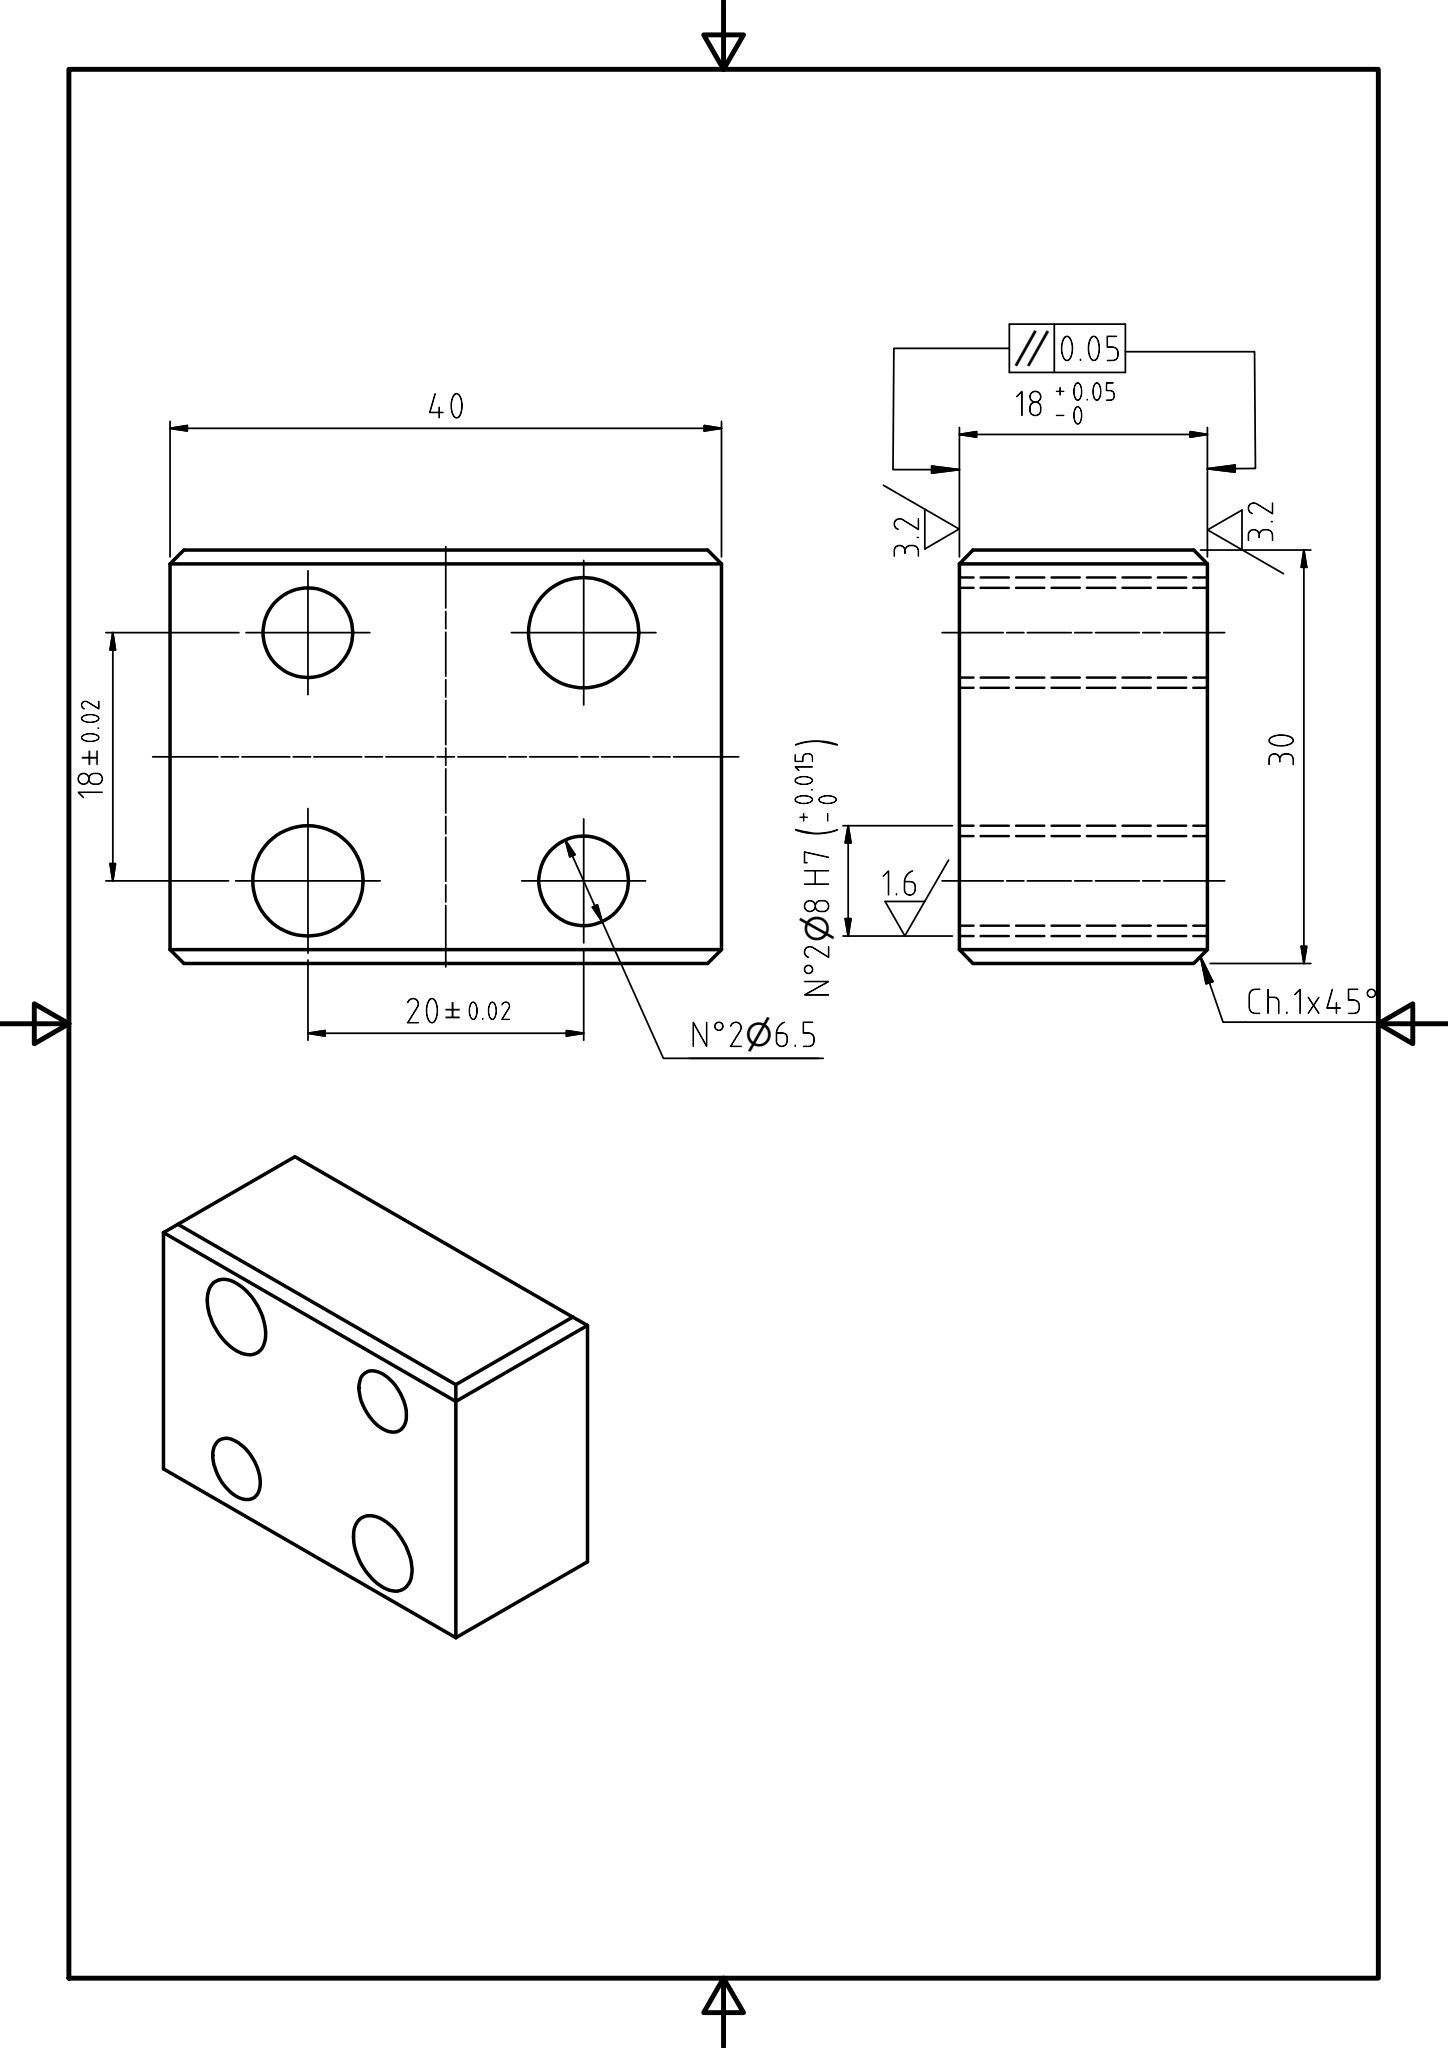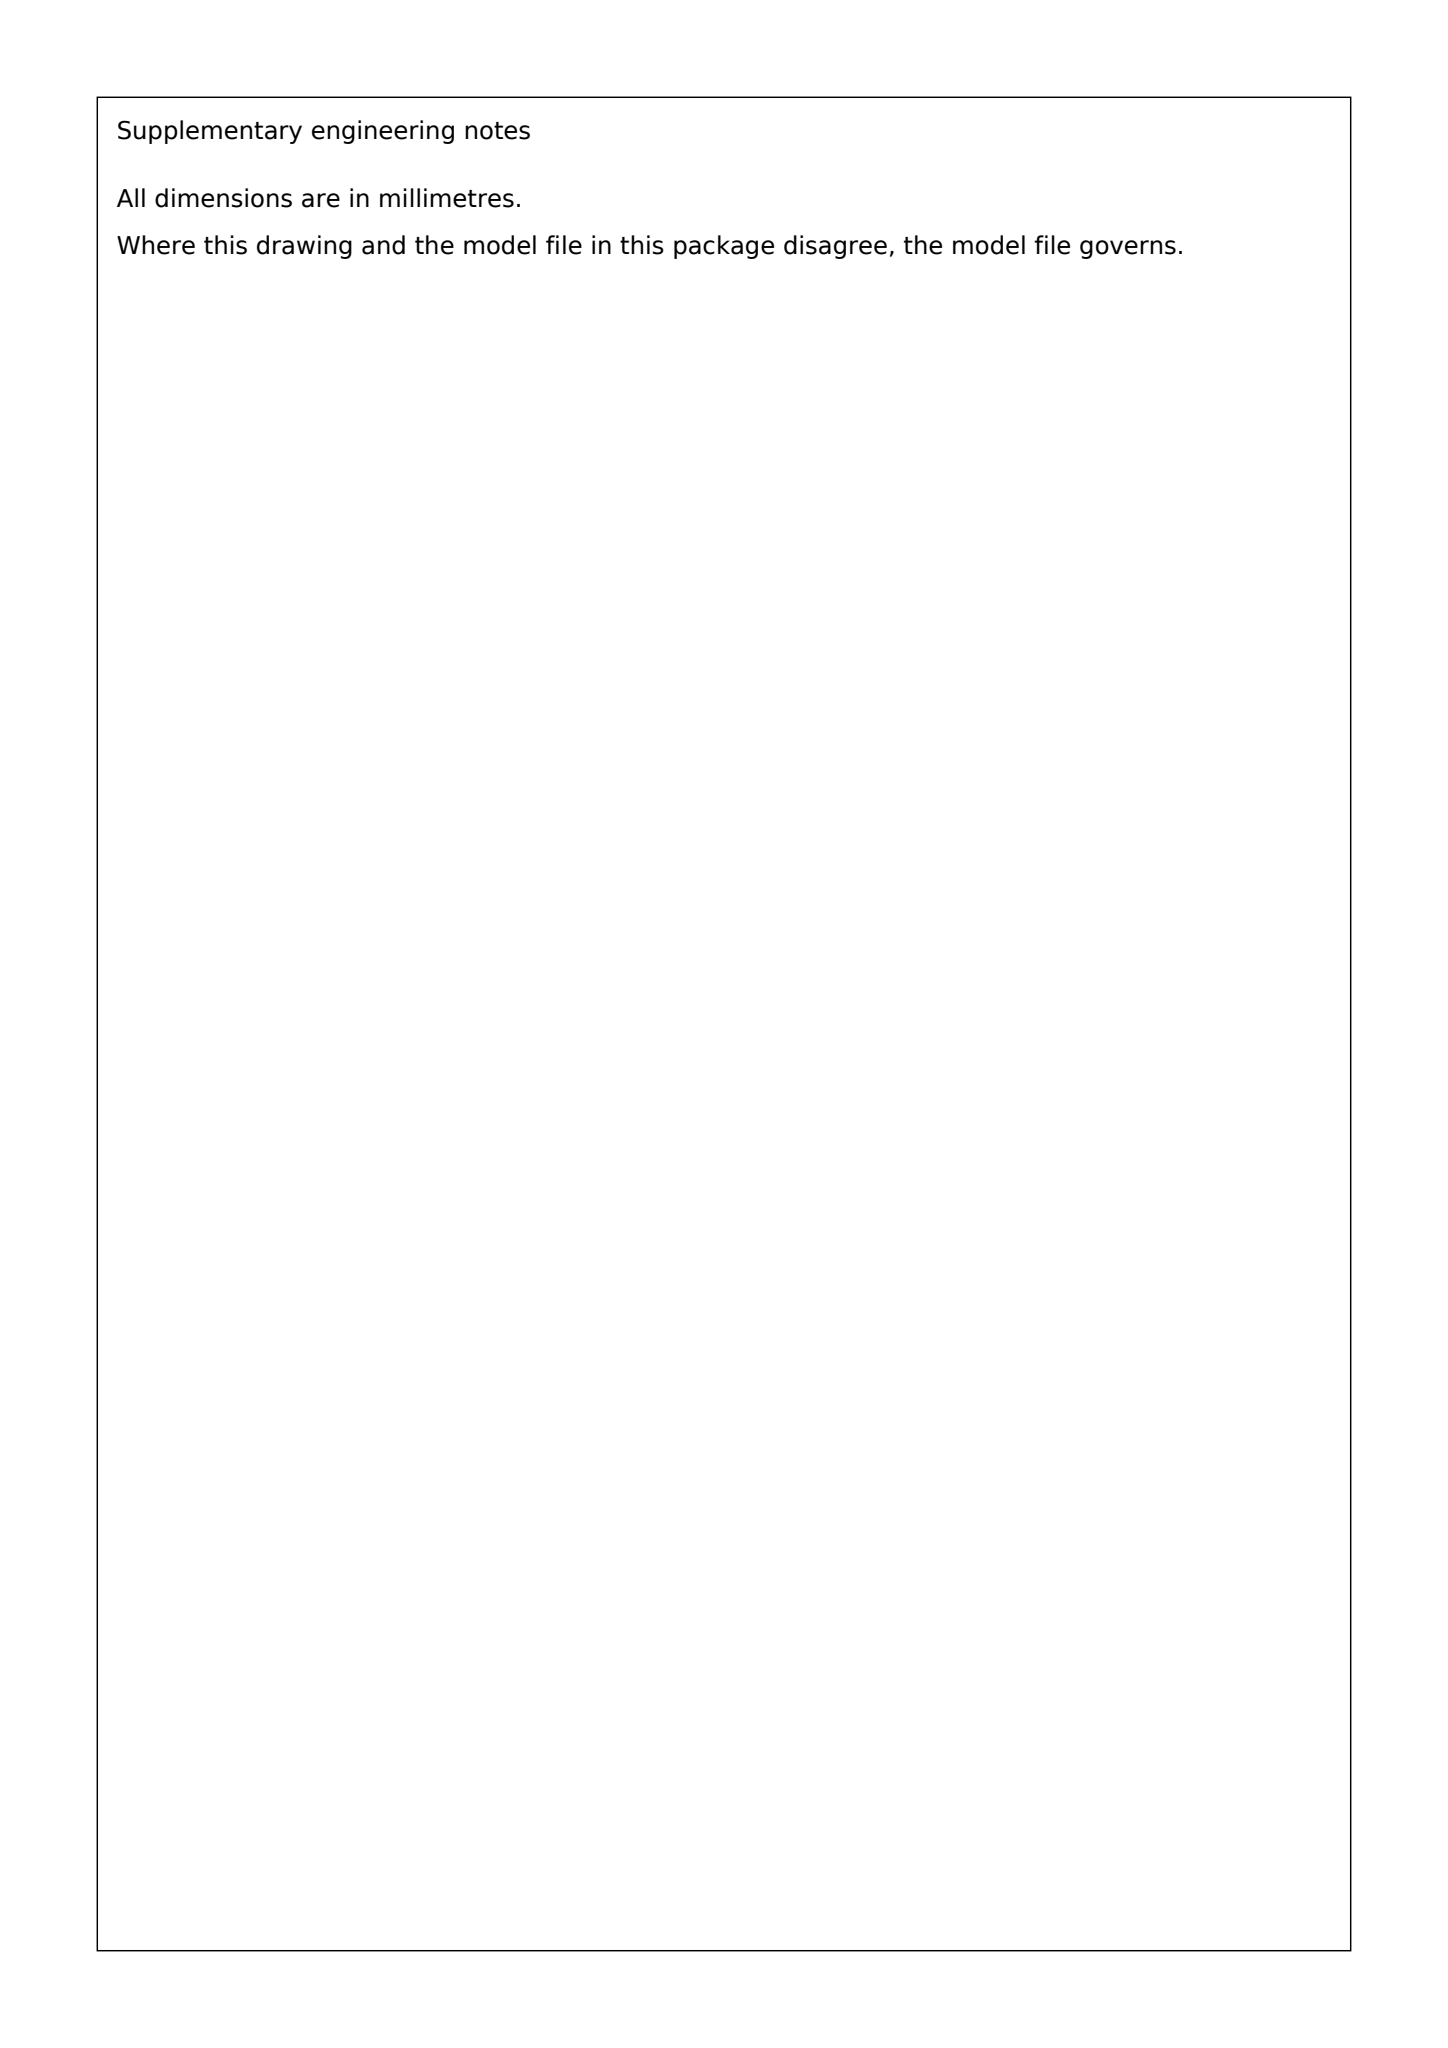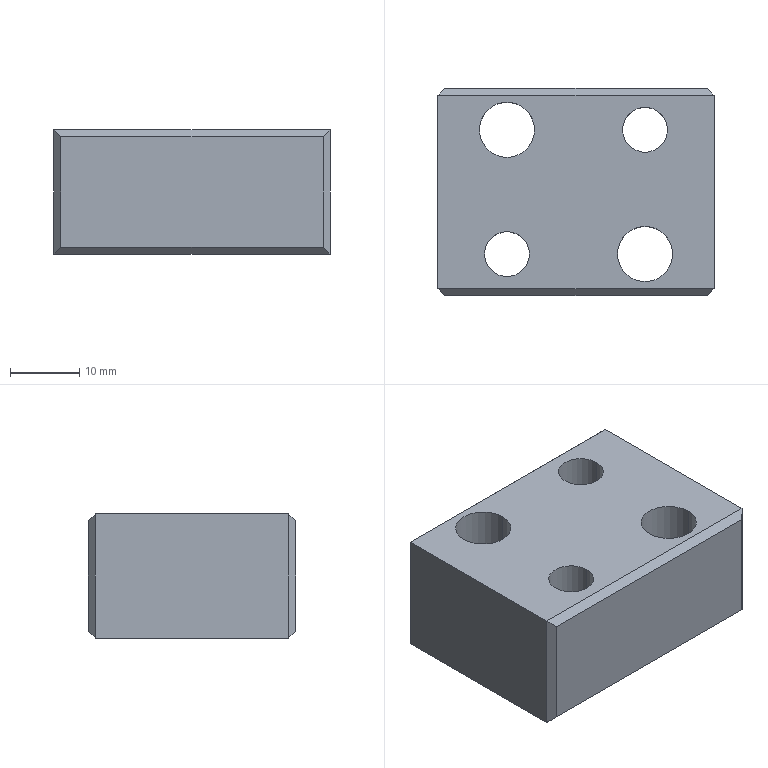Part | SolidWorks | mm | 1 solid | 22 faces | box 40 x 30 x 18 mm | volume 18483 mm3 | plane 14 | cylinder 8 | commonest cylinder face diameters 8 x4 6.5 x4
STEP:
#1=CARTESIAN_POINT('',(-14.,9.,-18.));
#2=VERTEX_POINT('',#1);
#3=CARTESIAN_POINT('',(-6.,9.,-18.));
#4=VERTEX_POINT('',#3);
#5=CARTESIAN_POINT('',(-10.,9.,-18.));
#6=DIRECTION('',(0.,0.,1.));
#7=DIRECTION('',(1.,0.,0.));
#8=AXIS2_PLACEMENT_3D('',#5,#6,#7);
#9=CIRCLE('',#8,4.);
#10=EDGE_CURVE('',#2,#4,#9,.T.);
#11=ORIENTED_EDGE('',*,*,#10,.F.);
#12=CARTESIAN_POINT('',(-14.,9.,0.));
#13=VERTEX_POINT('',#12);
#14=CARTESIAN_POINT('',(-14.,9.,-53.141));
#15=DIRECTION('',(0.,0.,1.));
#16=VECTOR('',#15,1000.);
#17=LINE('',#14,#16);
#18=EDGE_CURVE('',#2,#13,#17,.T.);
#19=ORIENTED_EDGE('',*,*,#18,.T.);
#20=CARTESIAN_POINT('',(-6.,9.,0.));
#21=VERTEX_POINT('',#20);
#22=CARTESIAN_POINT('',(-10.,9.,0.));
#23=DIRECTION('',(0.,0.,-1.));
#24=DIRECTION('',(1.,0.,0.));
#25=AXIS2_PLACEMENT_3D('',#22,#23,#24);
#26=CIRCLE('',#25,4.);
#27=EDGE_CURVE('',#21,#13,#26,.T.);
#28=ORIENTED_EDGE('',*,*,#27,.F.);
#29=CARTESIAN_POINT('',(-6.,9.,-53.141));
#30=DIRECTION('',(0.,0.,1.));
#31=VECTOR('',#30,1000.);
#32=LINE('',#29,#31);
#33=EDGE_CURVE('',#4,#21,#32,.T.);
#34=ORIENTED_EDGE('',*,*,#33,.F.);
#35=EDGE_LOOP('',(#11,#19,#28,#34));
#36=FACE_OUTER_BOUND('',#35,.T.);
#37=CARTESIAN_POINT('',(-10.,9.,-53.141));
#38=DIRECTION('',(0.,0.,1.));
#39=DIRECTION('',(1.,0.,0.));
#40=AXIS2_PLACEMENT_3D('',#37,#38,#39);
#41=CYLINDRICAL_SURFACE('',#40,4.);
#42=ADVANCED_FACE('',(#36),#41,.F.);
#43=CARTESIAN_POINT('',(6.,-9.,-18.));
#44=VERTEX_POINT('',#43);
#45=CARTESIAN_POINT('',(14.,-9.,-18.));
#46=VERTEX_POINT('',#45);
#47=CARTESIAN_POINT('',(10.,-9.,-18.));
#48=DIRECTION('',(0.,0.,1.));
#49=DIRECTION('',(1.,0.,0.));
#50=AXIS2_PLACEMENT_3D('',#47,#48,#49);
#51=CIRCLE('',#50,4.);
#52=EDGE_CURVE('',#44,#46,#51,.T.);
#53=ORIENTED_EDGE('',*,*,#52,.F.);
#54=CARTESIAN_POINT('',(6.,-9.,0.));
#55=VERTEX_POINT('',#54);
#56=CARTESIAN_POINT('',(6.,-9.,-53.141));
#57=DIRECTION('',(0.,0.,1.));
#58=VECTOR('',#57,1000.);
#59=LINE('',#56,#58);
#60=EDGE_CURVE('',#44,#55,#59,.T.);
#61=ORIENTED_EDGE('',*,*,#60,.T.);
#62=CARTESIAN_POINT('',(14.,-9.,0.));
#63=VERTEX_POINT('',#62);
#64=CARTESIAN_POINT('',(10.,-9.,0.));
#65=DIRECTION('',(0.,0.,-1.));
#66=DIRECTION('',(1.,0.,0.));
#67=AXIS2_PLACEMENT_3D('',#64,#65,#66);
#68=CIRCLE('',#67,4.);
#69=EDGE_CURVE('',#63,#55,#68,.T.);
#70=ORIENTED_EDGE('',*,*,#69,.F.);
#71=CARTESIAN_POINT('',(14.,-9.,-53.141));
#72=DIRECTION('',(0.,0.,1.));
#73=VECTOR('',#72,1000.);
#74=LINE('',#71,#73);
#75=EDGE_CURVE('',#46,#63,#74,.T.);
#76=ORIENTED_EDGE('',*,*,#75,.F.);
#77=EDGE_LOOP('',(#53,#61,#70,#76));
#78=FACE_OUTER_BOUND('',#77,.T.);
#79=CARTESIAN_POINT('',(10.,-9.,-53.141));
#80=DIRECTION('',(0.,0.,1.));
#81=DIRECTION('',(1.,0.,0.));
#82=AXIS2_PLACEMENT_3D('',#79,#80,#81);
#83=CYLINDRICAL_SURFACE('',#82,4.);
#84=ADVANCED_FACE('',(#78),#83,.F.);
#85=CARTESIAN_POINT('',(-13.25,-9.,-18.));
#86=VERTEX_POINT('',#85);
#87=CARTESIAN_POINT('',(-6.75,-9.,-18.));
#88=VERTEX_POINT('',#87);
#89=CARTESIAN_POINT('',(-10.,-9.,-18.));
#90=DIRECTION('',(0.,0.,1.));
#91=DIRECTION('',(1.,0.,0.));
#92=AXIS2_PLACEMENT_3D('',#89,#90,#91);
#93=CIRCLE('',#92,3.25);
#94=EDGE_CURVE('',#86,#88,#93,.T.);
#95=ORIENTED_EDGE('',*,*,#94,.F.);
#96=CARTESIAN_POINT('',(-13.25,-9.,0.));
#97=VERTEX_POINT('',#96);
#98=CARTESIAN_POINT('',(-13.25,-9.,-53.141));
#99=DIRECTION('',(0.,0.,1.));
#100=VECTOR('',#99,1000.);
#101=LINE('',#98,#100);
#102=EDGE_CURVE('',#86,#97,#101,.T.);
#103=ORIENTED_EDGE('',*,*,#102,.T.);
#104=CARTESIAN_POINT('',(-6.75,-9.,0.));
#105=VERTEX_POINT('',#104);
#106=CARTESIAN_POINT('',(-10.,-9.,0.));
#107=DIRECTION('',(0.,0.,-1.));
#108=DIRECTION('',(1.,0.,0.));
#109=AXIS2_PLACEMENT_3D('',#106,#107,#108);
#110=CIRCLE('',#109,3.25);
#111=EDGE_CURVE('',#105,#97,#110,.T.);
#112=ORIENTED_EDGE('',*,*,#111,.F.);
#113=CARTESIAN_POINT('',(-6.75,-9.,-53.141));
#114=DIRECTION('',(0.,0.,1.));
#115=VECTOR('',#114,1000.);
#116=LINE('',#113,#115);
#117=EDGE_CURVE('',#88,#105,#116,.T.);
#118=ORIENTED_EDGE('',*,*,#117,.F.);
#119=EDGE_LOOP('',(#95,#103,#112,#118));
#120=FACE_OUTER_BOUND('',#119,.T.);
#121=CARTESIAN_POINT('',(-10.,-9.,-53.141));
#122=DIRECTION('',(0.,0.,1.));
#123=DIRECTION('',(1.,0.,0.));
#124=AXIS2_PLACEMENT_3D('',#121,#122,#123);
#125=CYLINDRICAL_SURFACE('',#124,3.25);
#126=ADVANCED_FACE('',(#120),#125,.F.);
#127=CARTESIAN_POINT('',(6.75,9.,-18.));
#128=VERTEX_POINT('',#127);
#129=CARTESIAN_POINT('',(13.25,9.,-18.));
#130=VERTEX_POINT('',#129);
#131=CARTESIAN_POINT('',(10.,9.,-18.));
#132=DIRECTION('',(0.,0.,1.));
#133=DIRECTION('',(1.,0.,0.));
#134=AXIS2_PLACEMENT_3D('',#131,#132,#133);
#135=CIRCLE('',#134,3.25);
#136=EDGE_CURVE('',#128,#130,#135,.T.);
#137=ORIENTED_EDGE('',*,*,#136,.F.);
#138=CARTESIAN_POINT('',(6.75,9.,0.));
#139=VERTEX_POINT('',#138);
#140=CARTESIAN_POINT('',(6.75,9.,-53.141));
#141=DIRECTION('',(0.,0.,1.));
#142=VECTOR('',#141,1000.);
#143=LINE('',#140,#142);
#144=EDGE_CURVE('',#128,#139,#143,.T.);
#145=ORIENTED_EDGE('',*,*,#144,.T.);
#146=CARTESIAN_POINT('',(13.25,9.,0.));
#147=VERTEX_POINT('',#146);
#148=CARTESIAN_POINT('',(10.,9.,0.));
#149=DIRECTION('',(0.,0.,-1.));
#150=DIRECTION('',(1.,0.,0.));
#151=AXIS2_PLACEMENT_3D('',#148,#149,#150);
#152=CIRCLE('',#151,3.25);
#153=EDGE_CURVE('',#147,#139,#152,.T.);
#154=ORIENTED_EDGE('',*,*,#153,.F.);
#155=CARTESIAN_POINT('',(13.25,9.,-53.141));
#156=DIRECTION('',(0.,0.,1.));
#157=VECTOR('',#156,1000.);
#158=LINE('',#155,#157);
#159=EDGE_CURVE('',#130,#147,#158,.T.);
#160=ORIENTED_EDGE('',*,*,#159,.F.);
#161=EDGE_LOOP('',(#137,#145,#154,#160));
#162=FACE_OUTER_BOUND('',#161,.T.);
#163=CARTESIAN_POINT('',(10.,9.,-53.141));
#164=DIRECTION('',(0.,0.,1.));
#165=DIRECTION('',(1.,0.,0.));
#166=AXIS2_PLACEMENT_3D('',#163,#164,#165);
#167=CYLINDRICAL_SURFACE('',#166,3.25);
#168=ADVANCED_FACE('',(#162),#167,.F.);
#169=CARTESIAN_POINT('',(20.,-14.,0.));
#170=VERTEX_POINT('',#169);
#171=CARTESIAN_POINT('',(-20.,-14.,0.));
#172=VERTEX_POINT('',#171);
#173=CARTESIAN_POINT('',(-10.,-14.,0.));
#174=DIRECTION('',(-1.,-0.,0.));
#175=VECTOR('',#174,1000.);
#176=LINE('',#173,#175);
#177=EDGE_CURVE('',#170,#172,#176,.T.);
#178=ORIENTED_EDGE('',*,*,#177,.T.);
#179=CARTESIAN_POINT('',(-19.,-15.,-1.));
#180=VERTEX_POINT('',#179);
#181=CARTESIAN_POINT('',(-20.,-14.,0.));
#182=DIRECTION('',(0.5774,-0.5774,-0.5774));
#183=VECTOR('',#182,1000.);
#184=LINE('',#181,#183);
#185=EDGE_CURVE('',#172,#180,#184,.T.);
#186=ORIENTED_EDGE('',*,*,#185,.T.);
#187=CARTESIAN_POINT('',(19.,-15.,-1.));
#188=VERTEX_POINT('',#187);
#189=CARTESIAN_POINT('',(-10.,-15.,-1.));
#190=DIRECTION('',(1.,0.,0.));
#191=VECTOR('',#190,1000.);
#192=LINE('',#189,#191);
#193=EDGE_CURVE('',#180,#188,#192,.T.);
#194=ORIENTED_EDGE('',*,*,#193,.T.);
#195=CARTESIAN_POINT('',(19.,-15.,-1.));
#196=DIRECTION('',(0.5774,0.5774,0.5774));
#197=VECTOR('',#196,1000.);
#198=LINE('',#195,#197);
#199=EDGE_CURVE('',#188,#170,#198,.T.);
#200=ORIENTED_EDGE('',*,*,#199,.T.);
#201=EDGE_LOOP('',(#178,#186,#194,#200));
#202=FACE_OUTER_BOUND('',#201,.T.);
#203=CARTESIAN_POINT('',(-10.,-14.5,-0.5));
#204=DIRECTION('',(0.,-0.7071,0.7071));
#205=DIRECTION('',(-1.,-0.,0.));
#206=AXIS2_PLACEMENT_3D('',#203,#204,#205);
#207=PLANE('',#206);
#208=ADVANCED_FACE('',(#202),#207,.T.);
#209=CARTESIAN_POINT('',(19.,-15.,-17.));
#210=VERTEX_POINT('',#209);
#211=CARTESIAN_POINT('',(19.,-15.,0.));
#212=DIRECTION('',(0.,0.,-1.));
#213=VECTOR('',#212,1000.);
#214=LINE('',#211,#213);
#215=EDGE_CURVE('',#188,#210,#214,.T.);
#216=ORIENTED_EDGE('',*,*,#215,.T.);
#217=CARTESIAN_POINT('',(20.,-14.,-18.));
#218=VERTEX_POINT('',#217);
#219=CARTESIAN_POINT('',(19.,-15.,-17.));
#220=DIRECTION('',(0.5774,0.5774,-0.5774));
#221=VECTOR('',#220,1000.);
#222=LINE('',#219,#221);
#223=EDGE_CURVE('',#210,#218,#222,.T.);
#224=ORIENTED_EDGE('',*,*,#223,.T.);
#225=CARTESIAN_POINT('',(20.,-14.,0.));
#226=DIRECTION('',(0.,0.,1.));
#227=VECTOR('',#226,1000.);
#228=LINE('',#225,#227);
#229=EDGE_CURVE('',#218,#170,#228,.T.);
#230=ORIENTED_EDGE('',*,*,#229,.T.);
#231=ORIENTED_EDGE('',*,*,#199,.F.);
#232=EDGE_LOOP('',(#216,#224,#230,#231));
#233=FACE_OUTER_BOUND('',#232,.T.);
#234=CARTESIAN_POINT('',(19.5,-14.5,0.));
#235=DIRECTION('',(0.7071,-0.7071,0.));
#236=DIRECTION('',(0.,0.,-1.));
#237=AXIS2_PLACEMENT_3D('',#234,#235,#236);
#238=PLANE('',#237);
#239=ADVANCED_FACE('',(#233),#238,.T.);
#240=CARTESIAN_POINT('',(-20.,-14.,-18.));
#241=VERTEX_POINT('',#240);
#242=CARTESIAN_POINT('',(-10.,-14.,-18.));
#243=DIRECTION('',(1.,0.,0.));
#244=VECTOR('',#243,1000.);
#245=LINE('',#242,#244);
#246=EDGE_CURVE('',#241,#218,#245,.T.);
#247=ORIENTED_EDGE('',*,*,#246,.T.);
#248=ORIENTED_EDGE('',*,*,#223,.F.);
#249=CARTESIAN_POINT('',(-19.,-15.,-17.));
#250=VERTEX_POINT('',#249);
#251=CARTESIAN_POINT('',(-10.,-15.,-17.));
#252=DIRECTION('',(-1.,-0.,0.));
#253=VECTOR('',#252,1000.);
#254=LINE('',#251,#253);
#255=EDGE_CURVE('',#210,#250,#254,.T.);
#256=ORIENTED_EDGE('',*,*,#255,.T.);
#257=CARTESIAN_POINT('',(-20.,-14.,-18.));
#258=DIRECTION('',(0.5774,-0.5774,0.5774));
#259=VECTOR('',#258,1000.);
#260=LINE('',#257,#259);
#261=EDGE_CURVE('',#241,#250,#260,.T.);
#262=ORIENTED_EDGE('',*,*,#261,.F.);
#263=EDGE_LOOP('',(#247,#248,#256,#262));
#264=FACE_OUTER_BOUND('',#263,.T.);
#265=CARTESIAN_POINT('',(-10.,-14.5,-17.5));
#266=DIRECTION('',(0.,-0.7071,-0.7071));
#267=DIRECTION('',(0.,-0.7071,0.7071));
#268=AXIS2_PLACEMENT_3D('',#265,#266,#267);
#269=PLANE('',#268);
#270=ADVANCED_FACE('',(#264),#269,.T.);
#271=CARTESIAN_POINT('',(-20.,-14.,0.));
#272=DIRECTION('',(0.,0.,-1.));
#273=VECTOR('',#272,1000.);
#274=LINE('',#271,#273);
#275=EDGE_CURVE('',#172,#241,#274,.T.);
#276=ORIENTED_EDGE('',*,*,#275,.T.);
#277=ORIENTED_EDGE('',*,*,#261,.T.);
#278=CARTESIAN_POINT('',(-19.,-15.,0.));
#279=DIRECTION('',(0.,0.,1.));
#280=VECTOR('',#279,1000.);
#281=LINE('',#278,#280);
#282=EDGE_CURVE('',#250,#180,#281,.T.);
#283=ORIENTED_EDGE('',*,*,#282,.T.);
#284=ORIENTED_EDGE('',*,*,#185,.F.);
#285=EDGE_LOOP('',(#276,#277,#283,#284));
#286=FACE_OUTER_BOUND('',#285,.T.);
#287=CARTESIAN_POINT('',(-19.5,-14.5,0.));
#288=DIRECTION('',(-0.7071,-0.7071,0.));
#289=DIRECTION('',(-0.7071,0.7071,0.));
#290=AXIS2_PLACEMENT_3D('',#287,#288,#289);
#291=PLANE('',#290);
#292=ADVANCED_FACE('',(#286),#291,.T.);
#293=ORIENTED_EDGE('',*,*,#275,.F.);
#294=CARTESIAN_POINT('',(-20.,14.,0.));
#295=VERTEX_POINT('',#294);
#296=CARTESIAN_POINT('',(-20.,-15.,0.));
#297=DIRECTION('',(0.,1.,0.));
#298=VECTOR('',#297,1000.);
#299=LINE('',#296,#298);
#300=EDGE_CURVE('',#172,#295,#299,.T.);
#301=ORIENTED_EDGE('',*,*,#300,.T.);
#302=CARTESIAN_POINT('',(-20.,14.,-18.));
#303=VERTEX_POINT('',#302);
#304=CARTESIAN_POINT('',(-20.,14.,0.));
#305=DIRECTION('',(0.,0.,1.));
#306=VECTOR('',#305,1000.);
#307=LINE('',#304,#306);
#308=EDGE_CURVE('',#303,#295,#307,.T.);
#309=ORIENTED_EDGE('',*,*,#308,.F.);
#310=CARTESIAN_POINT('',(-20.,-15.,-18.));
#311=DIRECTION('',(0.,-1.,0.));
#312=VECTOR('',#311,1000.);
#313=LINE('',#310,#312);
#314=EDGE_CURVE('',#303,#241,#313,.T.);
#315=ORIENTED_EDGE('',*,*,#314,.T.);
#316=EDGE_LOOP('',(#293,#301,#309,#315));
#317=FACE_OUTER_BOUND('',#316,.T.);
#318=CARTESIAN_POINT('',(-20.,15.,0.));
#319=DIRECTION('',(-1.,0.,0.));
#320=DIRECTION('',(0.,0.,1.));
#321=AXIS2_PLACEMENT_3D('',#318,#319,#320);
#322=PLANE('',#321);
#323=ADVANCED_FACE('',(#317),#322,.T.);
#324=ORIENTED_EDGE('',*,*,#177,.F.);
#325=CARTESIAN_POINT('',(20.,14.,0.));
#326=VERTEX_POINT('',#325);
#327=CARTESIAN_POINT('',(20.,15.,0.));
#328=DIRECTION('',(0.,-1.,0.));
#329=VECTOR('',#328,1000.);
#330=LINE('',#327,#329);
#331=EDGE_CURVE('',#326,#170,#330,.T.);
#332=ORIENTED_EDGE('',*,*,#331,.F.);
#333=CARTESIAN_POINT('',(10.,14.,0.));
#334=DIRECTION('',(1.,-0.,0.));
#335=VECTOR('',#334,1000.);
#336=LINE('',#333,#335);
#337=EDGE_CURVE('',#295,#326,#336,.T.);
#338=ORIENTED_EDGE('',*,*,#337,.F.);
#339=ORIENTED_EDGE('',*,*,#300,.F.);
#340=EDGE_LOOP('',(#324,#332,#338,#339));
#341=FACE_OUTER_BOUND('',#340,.T.);
#342=ORIENTED_EDGE('',*,*,#153,.T.);
#343=CARTESIAN_POINT('',(10.,9.,0.));
#344=DIRECTION('',(0.,0.,-1.));
#345=DIRECTION('',(1.,0.,0.));
#346=AXIS2_PLACEMENT_3D('',#343,#344,#345);
#347=CIRCLE('',#346,3.25);
#348=EDGE_CURVE('',#139,#147,#347,.T.);
#349=ORIENTED_EDGE('',*,*,#348,.T.);
#350=EDGE_LOOP('',(#342,#349));
#351=FACE_BOUND('',#350,.T.);
#352=ORIENTED_EDGE('',*,*,#111,.T.);
#353=CARTESIAN_POINT('',(-10.,-9.,0.));
#354=DIRECTION('',(0.,0.,-1.));
#355=DIRECTION('',(1.,0.,0.));
#356=AXIS2_PLACEMENT_3D('',#353,#354,#355);
#357=CIRCLE('',#356,3.25);
#358=EDGE_CURVE('',#97,#105,#357,.T.);
#359=ORIENTED_EDGE('',*,*,#358,.T.);
#360=EDGE_LOOP('',(#352,#359));
#361=FACE_BOUND('',#360,.T.);
#362=ORIENTED_EDGE('',*,*,#69,.T.);
#363=CARTESIAN_POINT('',(10.,-9.,0.));
#364=DIRECTION('',(0.,0.,-1.));
#365=DIRECTION('',(1.,0.,0.));
#366=AXIS2_PLACEMENT_3D('',#363,#364,#365);
#367=CIRCLE('',#366,4.);
#368=EDGE_CURVE('',#55,#63,#367,.T.);
#369=ORIENTED_EDGE('',*,*,#368,.T.);
#370=EDGE_LOOP('',(#362,#369));
#371=FACE_BOUND('',#370,.T.);
#372=ORIENTED_EDGE('',*,*,#27,.T.);
#373=CARTESIAN_POINT('',(-10.,9.,0.));
#374=DIRECTION('',(0.,0.,-1.));
#375=DIRECTION('',(1.,0.,0.));
#376=AXIS2_PLACEMENT_3D('',#373,#374,#375);
#377=CIRCLE('',#376,4.);
#378=EDGE_CURVE('',#13,#21,#377,.T.);
#379=ORIENTED_EDGE('',*,*,#378,.T.);
#380=EDGE_LOOP('',(#372,#379));
#381=FACE_BOUND('',#380,.T.);
#382=CARTESIAN_POINT('',(0.,0.,0.));
#383=DIRECTION('',(0.,0.,1.));
#384=DIRECTION('',(1.,0.,0.));
#385=AXIS2_PLACEMENT_3D('',#382,#383,#384);
#386=PLANE('',#385);
#387=ADVANCED_FACE('',(#341,#351,#361,#371,#381),#386,.T.);
#388=ORIENTED_EDGE('',*,*,#193,.F.);
#389=ORIENTED_EDGE('',*,*,#282,.F.);
#390=ORIENTED_EDGE('',*,*,#255,.F.);
#391=ORIENTED_EDGE('',*,*,#215,.F.);
#392=EDGE_LOOP('',(#388,#389,#390,#391));
#393=FACE_OUTER_BOUND('',#392,.T.);
#394=CARTESIAN_POINT('',(-20.,-15.,0.));
#395=DIRECTION('',(0.,-1.,0.));
#396=DIRECTION('',(0.,0.,-1.));
#397=AXIS2_PLACEMENT_3D('',#394,#395,#396);
#398=PLANE('',#397);
#399=ADVANCED_FACE('',(#393),#398,.T.);
#400=ORIENTED_EDGE('',*,*,#337,.T.);
#401=CARTESIAN_POINT('',(19.,15.,-1.));
#402=VERTEX_POINT('',#401);
#403=CARTESIAN_POINT('',(20.,14.,0.));
#404=DIRECTION('',(-0.5774,0.5774,-0.5774));
#405=VECTOR('',#404,1000.);
#406=LINE('',#403,#405);
#407=EDGE_CURVE('',#326,#402,#406,.T.);
#408=ORIENTED_EDGE('',*,*,#407,.T.);
#409=CARTESIAN_POINT('',(-19.,15.,-1.));
#410=VERTEX_POINT('',#409);
#411=CARTESIAN_POINT('',(10.,15.,-1.));
#412=DIRECTION('',(-1.,0.,0.));
#413=VECTOR('',#412,1000.);
#414=LINE('',#411,#413);
#415=EDGE_CURVE('',#402,#410,#414,.T.);
#416=ORIENTED_EDGE('',*,*,#415,.T.);
#417=CARTESIAN_POINT('',(-19.,15.,-1.));
#418=DIRECTION('',(-0.5774,-0.5774,0.5774));
#419=VECTOR('',#418,1000.);
#420=LINE('',#417,#419);
#421=EDGE_CURVE('',#410,#295,#420,.T.);
#422=ORIENTED_EDGE('',*,*,#421,.T.);
#423=EDGE_LOOP('',(#400,#408,#416,#422));
#424=FACE_OUTER_BOUND('',#423,.T.);
#425=CARTESIAN_POINT('',(10.,14.5,-0.5));
#426=DIRECTION('',(0.,0.7071,0.7071));
#427=DIRECTION('',(1.,-0.,0.));
#428=AXIS2_PLACEMENT_3D('',#425,#426,#427);
#429=PLANE('',#428);
#430=ADVANCED_FACE('',(#424),#429,.T.);
#431=CARTESIAN_POINT('',(-19.,15.,-17.));
#432=VERTEX_POINT('',#431);
#433=CARTESIAN_POINT('',(-19.,15.,0.));
#434=DIRECTION('',(0.,0.,-1.));
#435=VECTOR('',#434,1000.);
#436=LINE('',#433,#435);
#437=EDGE_CURVE('',#410,#432,#436,.T.);
#438=ORIENTED_EDGE('',*,*,#437,.T.);
#439=CARTESIAN_POINT('',(-19.,15.,-17.));
#440=DIRECTION('',(-0.5774,-0.5774,-0.5774));
#441=VECTOR('',#440,1000.);
#442=LINE('',#439,#441);
#443=EDGE_CURVE('',#432,#303,#442,.T.);
#444=ORIENTED_EDGE('',*,*,#443,.T.);
#445=ORIENTED_EDGE('',*,*,#308,.T.);
#446=ORIENTED_EDGE('',*,*,#421,.F.);
#447=EDGE_LOOP('',(#438,#444,#445,#446));
#448=FACE_OUTER_BOUND('',#447,.T.);
#449=CARTESIAN_POINT('',(-19.5,14.5,0.));
#450=DIRECTION('',(-0.7071,0.7071,0.));
#451=DIRECTION('',(0.,0.,1.));
#452=AXIS2_PLACEMENT_3D('',#449,#450,#451);
#453=PLANE('',#452);
#454=ADVANCED_FACE('',(#448),#453,.T.);
#455=CARTESIAN_POINT('',(20.,14.,-18.));
#456=VERTEX_POINT('',#455);
#457=CARTESIAN_POINT('',(10.,14.,-18.));
#458=DIRECTION('',(-1.,0.,0.));
#459=VECTOR('',#458,1000.);
#460=LINE('',#457,#459);
#461=EDGE_CURVE('',#456,#303,#460,.T.);
#462=ORIENTED_EDGE('',*,*,#461,.T.);
#463=ORIENTED_EDGE('',*,*,#443,.F.);
#464=CARTESIAN_POINT('',(19.,15.,-17.));
#465=VERTEX_POINT('',#464);
#466=CARTESIAN_POINT('',(10.,15.,-17.));
#467=DIRECTION('',(1.,-0.,0.));
#468=VECTOR('',#467,1000.);
#469=LINE('',#466,#468);
#470=EDGE_CURVE('',#432,#465,#469,.T.);
#471=ORIENTED_EDGE('',*,*,#470,.T.);
#472=CARTESIAN_POINT('',(20.,14.,-18.));
#473=DIRECTION('',(-0.5774,0.5774,0.5774));
#474=VECTOR('',#473,1000.);
#475=LINE('',#472,#474);
#476=EDGE_CURVE('',#456,#465,#475,.T.);
#477=ORIENTED_EDGE('',*,*,#476,.F.);
#478=EDGE_LOOP('',(#462,#463,#471,#477));
#479=FACE_OUTER_BOUND('',#478,.T.);
#480=CARTESIAN_POINT('',(10.,14.5,-17.5));
#481=DIRECTION('',(0.,0.7071,-0.7071));
#482=DIRECTION('',(-1.,0.,-0.));
#483=AXIS2_PLACEMENT_3D('',#480,#481,#482);
#484=PLANE('',#483);
#485=ADVANCED_FACE('',(#479),#484,.T.);
#486=CARTESIAN_POINT('',(20.,14.,0.));
#487=DIRECTION('',(0.,0.,-1.));
#488=VECTOR('',#487,1000.);
#489=LINE('',#486,#488);
#490=EDGE_CURVE('',#326,#456,#489,.T.);
#491=ORIENTED_EDGE('',*,*,#490,.T.);
#492=ORIENTED_EDGE('',*,*,#476,.T.);
#493=CARTESIAN_POINT('',(19.,15.,0.));
#494=DIRECTION('',(0.,0.,1.));
#495=VECTOR('',#494,1000.);
#496=LINE('',#493,#495);
#497=EDGE_CURVE('',#465,#402,#496,.T.);
#498=ORIENTED_EDGE('',*,*,#497,.T.);
#499=ORIENTED_EDGE('',*,*,#407,.F.);
#500=EDGE_LOOP('',(#491,#492,#498,#499));
#501=FACE_OUTER_BOUND('',#500,.T.);
#502=CARTESIAN_POINT('',(19.5,14.5,0.));
#503=DIRECTION('',(0.7071,0.7071,0.));
#504=DIRECTION('',(0.,0.,-1.));
#505=AXIS2_PLACEMENT_3D('',#502,#503,#504);
#506=PLANE('',#505);
#507=ADVANCED_FACE('',(#501),#506,.T.);
#508=ORIENTED_EDGE('',*,*,#229,.F.);
#509=CARTESIAN_POINT('',(20.,15.,-18.));
#510=DIRECTION('',(0.,1.,0.));
#511=VECTOR('',#510,1000.);
#512=LINE('',#509,#511);
#513=EDGE_CURVE('',#218,#456,#512,.T.);
#514=ORIENTED_EDGE('',*,*,#513,.T.);
#515=ORIENTED_EDGE('',*,*,#490,.F.);
#516=ORIENTED_EDGE('',*,*,#331,.T.);
#517=EDGE_LOOP('',(#508,#514,#515,#516));
#518=FACE_OUTER_BOUND('',#517,.T.);
#519=CARTESIAN_POINT('',(20.,-15.,0.));
#520=DIRECTION('',(1.,0.,0.));
#521=DIRECTION('',(0.,1.,0.));
#522=AXIS2_PLACEMENT_3D('',#519,#520,#521);
#523=PLANE('',#522);
#524=ADVANCED_FACE('',(#518),#523,.T.);
#525=ORIENTED_EDGE('',*,*,#415,.F.);
#526=ORIENTED_EDGE('',*,*,#497,.F.);
#527=ORIENTED_EDGE('',*,*,#470,.F.);
#528=ORIENTED_EDGE('',*,*,#437,.F.);
#529=EDGE_LOOP('',(#525,#526,#527,#528));
#530=FACE_OUTER_BOUND('',#529,.T.);
#531=CARTESIAN_POINT('',(20.,15.,0.));
#532=DIRECTION('',(0.,1.,0.));
#533=DIRECTION('',(1.,0.,-0.));
#534=AXIS2_PLACEMENT_3D('',#531,#532,#533);
#535=PLANE('',#534);
#536=ADVANCED_FACE('',(#530),#535,.T.);
#537=ORIENTED_EDGE('',*,*,#144,.F.);
#538=CARTESIAN_POINT('',(10.,9.,-18.));
#539=DIRECTION('',(0.,0.,1.));
#540=DIRECTION('',(1.,0.,0.));
#541=AXIS2_PLACEMENT_3D('',#538,#539,#540);
#542=CIRCLE('',#541,3.25);
#543=EDGE_CURVE('',#130,#128,#542,.T.);
#544=ORIENTED_EDGE('',*,*,#543,.F.);
#545=ORIENTED_EDGE('',*,*,#159,.T.);
#546=ORIENTED_EDGE('',*,*,#348,.F.);
#547=EDGE_LOOP('',(#537,#544,#545,#546));
#548=FACE_OUTER_BOUND('',#547,.T.);
#549=CARTESIAN_POINT('',(10.,9.,-53.141));
#550=DIRECTION('',(0.,0.,1.));
#551=DIRECTION('',(1.,0.,0.));
#552=AXIS2_PLACEMENT_3D('',#549,#550,#551);
#553=CYLINDRICAL_SURFACE('',#552,3.25);
#554=ADVANCED_FACE('',(#548),#553,.F.);
#555=ORIENTED_EDGE('',*,*,#102,.F.);
#556=CARTESIAN_POINT('',(-10.,-9.,-18.));
#557=DIRECTION('',(0.,0.,1.));
#558=DIRECTION('',(1.,0.,0.));
#559=AXIS2_PLACEMENT_3D('',#556,#557,#558);
#560=CIRCLE('',#559,3.25);
#561=EDGE_CURVE('',#88,#86,#560,.T.);
#562=ORIENTED_EDGE('',*,*,#561,.F.);
#563=ORIENTED_EDGE('',*,*,#117,.T.);
#564=ORIENTED_EDGE('',*,*,#358,.F.);
#565=EDGE_LOOP('',(#555,#562,#563,#564));
#566=FACE_OUTER_BOUND('',#565,.T.);
#567=CARTESIAN_POINT('',(-10.,-9.,-53.141));
#568=DIRECTION('',(0.,0.,1.));
#569=DIRECTION('',(1.,0.,0.));
#570=AXIS2_PLACEMENT_3D('',#567,#568,#569);
#571=CYLINDRICAL_SURFACE('',#570,3.25);
#572=ADVANCED_FACE('',(#566),#571,.F.);
#573=ORIENTED_EDGE('',*,*,#60,.F.);
#574=CARTESIAN_POINT('',(10.,-9.,-18.));
#575=DIRECTION('',(0.,0.,1.));
#576=DIRECTION('',(1.,0.,0.));
#577=AXIS2_PLACEMENT_3D('',#574,#575,#576);
#578=CIRCLE('',#577,4.);
#579=EDGE_CURVE('',#46,#44,#578,.T.);
#580=ORIENTED_EDGE('',*,*,#579,.F.);
#581=ORIENTED_EDGE('',*,*,#75,.T.);
#582=ORIENTED_EDGE('',*,*,#368,.F.);
#583=EDGE_LOOP('',(#573,#580,#581,#582));
#584=FACE_OUTER_BOUND('',#583,.T.);
#585=CARTESIAN_POINT('',(10.,-9.,-53.141));
#586=DIRECTION('',(0.,0.,1.));
#587=DIRECTION('',(1.,0.,0.));
#588=AXIS2_PLACEMENT_3D('',#585,#586,#587);
#589=CYLINDRICAL_SURFACE('',#588,4.);
#590=ADVANCED_FACE('',(#584),#589,.F.);
#591=ORIENTED_EDGE('',*,*,#18,.F.);
#592=CARTESIAN_POINT('',(-10.,9.,-18.));
#593=DIRECTION('',(0.,0.,1.));
#594=DIRECTION('',(1.,0.,0.));
#595=AXIS2_PLACEMENT_3D('',#592,#593,#594);
#596=CIRCLE('',#595,4.);
#597=EDGE_CURVE('',#4,#2,#596,.T.);
#598=ORIENTED_EDGE('',*,*,#597,.F.);
#599=ORIENTED_EDGE('',*,*,#33,.T.);
#600=ORIENTED_EDGE('',*,*,#378,.F.);
#601=EDGE_LOOP('',(#591,#598,#599,#600));
#602=FACE_OUTER_BOUND('',#601,.T.);
#603=CARTESIAN_POINT('',(-10.,9.,-53.141));
#604=DIRECTION('',(0.,0.,1.));
#605=DIRECTION('',(1.,0.,0.));
#606=AXIS2_PLACEMENT_3D('',#603,#604,#605);
#607=CYLINDRICAL_SURFACE('',#606,4.);
#608=ADVANCED_FACE('',(#602),#607,.F.);
#609=ORIENTED_EDGE('',*,*,#246,.F.);
#610=ORIENTED_EDGE('',*,*,#314,.F.);
#611=ORIENTED_EDGE('',*,*,#461,.F.);
#612=ORIENTED_EDGE('',*,*,#513,.F.);
#613=EDGE_LOOP('',(#609,#610,#611,#612));
#614=FACE_OUTER_BOUND('',#613,.T.);
#615=ORIENTED_EDGE('',*,*,#543,.T.);
#616=ORIENTED_EDGE('',*,*,#136,.T.);
#617=EDGE_LOOP('',(#615,#616));
#618=FACE_BOUND('',#617,.T.);
#619=ORIENTED_EDGE('',*,*,#561,.T.);
#620=ORIENTED_EDGE('',*,*,#94,.T.);
#621=EDGE_LOOP('',(#619,#620));
#622=FACE_BOUND('',#621,.T.);
#623=ORIENTED_EDGE('',*,*,#579,.T.);
#624=ORIENTED_EDGE('',*,*,#52,.T.);
#625=EDGE_LOOP('',(#623,#624));
#626=FACE_BOUND('',#625,.T.);
#627=ORIENTED_EDGE('',*,*,#597,.T.);
#628=ORIENTED_EDGE('',*,*,#10,.T.);
#629=EDGE_LOOP('',(#627,#628));
#630=FACE_BOUND('',#629,.T.);
#631=CARTESIAN_POINT('',(0.,0.,-18.));
#632=DIRECTION('',(0.,0.,1.));
#633=DIRECTION('',(1.,0.,0.));
#634=AXIS2_PLACEMENT_3D('',#631,#632,#633);
#635=PLANE('',#634);
#636=ADVANCED_FACE('',(#614,#618,#622,#626,#630),#635,.F.);
#637=CLOSED_SHELL('',(#42,#84,#126,#168,#208,#239,#270,#292,#323,#387,#399,#430,#454,#485,#507,#524,#536,#554,#572,#590,#608,#636));
#638=MANIFOLD_SOLID_BREP('',#637);
#639=CARTESIAN_POINT('',(0.,0.,0.));
#640=DIRECTION('',(0.,0.,1.));
#641=DIRECTION('',(1.,0.,0.));
#642=AXIS2_PLACEMENT_3D('',#639,#640,#641);
#643=(LENGTH_UNIT()NAMED_UNIT(*)SI_UNIT(.MILLI.,.METRE.));
#644=UNCERTAINTY_MEASURE_WITH_UNIT(LENGTH_MEASURE(0.00001),#643,'','');
#645=(NAMED_UNIT(*)PLANE_ANGLE_UNIT()SI_UNIT($,.RADIAN.));
#646=(NAMED_UNIT(*)SI_UNIT($,.STERADIAN.)SOLID_ANGLE_UNIT());
#647=(GEOMETRIC_REPRESENTATION_CONTEXT(3)GLOBAL_UNCERTAINTY_ASSIGNED_CONTEXT((#644))GLOBAL_UNIT_ASSIGNED_CONTEXT((#643,#645,#646))REPRESENTATION_CONTEXT('',''));
#648=ADVANCED_BREP_SHAPE_REPRESENTATION('',(#638,#642),#647);